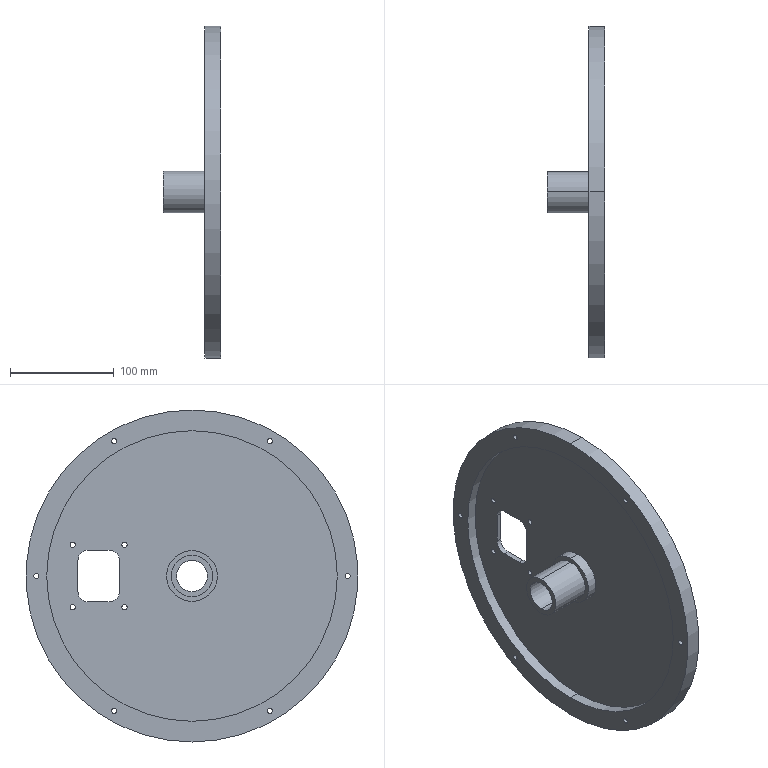Component | SolidWorks | SeedingAssemblyA-1_SeedingPlate-1 | 1 solid | 43 faces | box 55 x 320 x 320 mm | volume 609134 mm3 | cylinder 34 | plane 9 | commonest cylinder face diameters 5 x20 20 x4 49 x2 280 x2 30 x2 40 x2 320 x2
build123d program:
from build123d import *

# Parameters (mm, degrees)
SKETCH1_R             = 160
BOSS_EXTRUDE1_DEPTH   = 15
SKETCH2_R             = 20
BOSS_EXTRUDE2_DEPTH   = 40
SKETCH3_R             = 15
CUT_EXTRUDE1_DEPTH    = 233.863
SKETCH4_R             = 140
SKETCH4_R_2           = 24.5
CUT_EXTRUDE2_DEPTH    = 10
SKETCH5_W             = 50
SKETCH5_H             = 40
CUT_EXTRUDE3_DEPTH    = 233.863
FILLET1_R             = 10
SKETCH6_R             = 2.5
CUT_EXTRUDE4_DEPTH    = 233.863
CIRPATTERN1_COUNT     = 6
M6_TAPPED_HOLE1_D     = 5
M6_TAPPED_HOLE1_DEPTH = 17
M6_TAPPED_HOLE1_TIP   = 1.502


with BuildPart() as part:
    # Sketch1 → Boss-Extrude1 (new body)
    with BuildSketch(Plane.XY):
        Circle(SKETCH1_R)
    extrude(amount=BOSS_EXTRUDE1_DEPTH)

    # Sketch2 → Boss-Extrude2 (add)
    with BuildSketch(Plane.XY.offset(15)):
        Circle(SKETCH2_R)
    extrude(amount=BOSS_EXTRUDE2_DEPTH)

    # Sketch3 → Cut-Extrude1 (cut, through all)
    with BuildSketch(Plane.XY.offset(55)):
        Circle(SKETCH3_R)
    extrude(amount=-CUT_EXTRUDE1_DEPTH, mode=Mode.SUBTRACT)

    # Sketch4 → Cut-Extrude2 (cut)
    with BuildSketch(Plane.XY.offset(15)):
        Circle(SKETCH4_R)
        Circle(SKETCH4_R_2, mode=Mode.SUBTRACT)
    extrude(amount=-CUT_EXTRUDE2_DEPTH, mode=Mode.SUBTRACT)

    # Sketch5 → Cut-Extrude3 (cut, through all)
    with BuildSketch(Plane(origin=(0, 0, 0), x_dir=(-1, 0, 0), z_dir=(0, 0, -1))):
        with Locations((0, 90)):
            Rectangle(SKETCH5_W, SKETCH5_H)
    extrude(amount=-CUT_EXTRUDE3_DEPTH, mode=Mode.SUBTRACT)

    # Fillet1
    fillet1_edges = [part.edges().sort_by_distance(p)[0] for p in [
        (25, 70, 2.5),
        (25, 110, 2.5),
        (-25, 110, 2.5),
        (-25, 70, 2.5),
    ]]
    fillet(fillet1_edges, radius=FILLET1_R)

    # Sketch6 → Cut-Extrude4 (cut, through all)
    with BuildSketch(Plane(origin=(0, 0, 0), x_dir=(-1, 0, 0), z_dir=(0, 0, -1))):
        with Locations((0, 150)):
            Circle(SKETCH6_R)
    cut_extrude4 = extrude(amount=-CUT_EXTRUDE4_DEPTH, mode=Mode.SUBTRACT)

    # CirPattern1: Cut-Extrude4 ×6 about axis
    cirpattern1_axis = Axis((0, 0, 0), (0, 0, 1))
    for i in range(1, CIRPATTERN1_COUNT):
        add(cut_extrude4.rotate(cirpattern1_axis, i * 360 / CIRPATTERN1_COUNT), mode=Mode.SUBTRACT)

    # M6 Tapped Hole1
    with Locations(Plane(origin=(0, 0, 0), x_dir=(-1, 0, 0), z_dir=(0, 0, -1))):
        with Locations((-30, 65), (30, 65), (30, 115), (-30, 115)):
            Hole(M6_TAPPED_HOLE1_D / 2, depth=M6_TAPPED_HOLE1_DEPTH)
            with Locations((0, 0, -(M6_TAPPED_HOLE1_DEPTH + M6_TAPPED_HOLE1_TIP / 2))):  # 118° drill point
                Cone(0, M6_TAPPED_HOLE1_D / 2, M6_TAPPED_HOLE1_TIP, mode=Mode.SUBTRACT)


solid = part.part

# Placed as in the assembly
solid = solid.moved(Location((145.776, -105, -252.184), (0, -90, 0)))